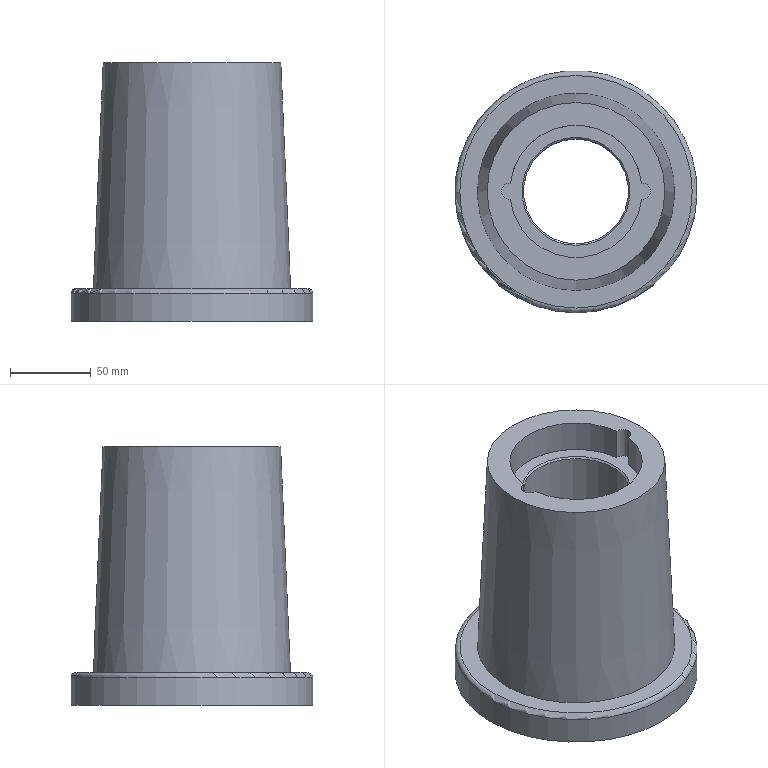Component | NX | BASE | 1 solid | 15 faces | box 150 x 150 x 160 mm | volume 816853 mm3 | cylinder 6 | plane 5 | cone 3 | torus 1 | commonest cylinder face diameters 82 x2 10 x2 150 x1 65 x1
STEP:
#1=CARTESIAN_POINT('',(0.,0.,0.));
#2=DIRECTION('',(0.,0.,1.));
#3=DIRECTION('',(1.,0.,0.));
#4=AXIS2_PLACEMENT_3D('',#1,#2,#3);
#5=CARTESIAN_POINT('',(-40.695,-4.991,140.));
#6=VERTEX_POINT('',#5);
#7=CARTESIAN_POINT('',(-40.695,-4.991,160.));
#8=VERTEX_POINT('',#7);
#9=CARTESIAN_POINT('',(-40.695,-4.991,150.));
#10=DIRECTION('',(0.,0.,1.));
#11=VECTOR('',#10,1.);
#12=LINE('',#9,#11);
#13=CARTESIAN_POINT('',(0.,0.,160.));
#14=DIRECTION('',(0.,0.,-1.));
#15=DIRECTION('',(0.,-1.,0.));
#16=AXIS2_PLACEMENT_3D('',#13,#14,#15);
#17=CYLINDRICAL_SURFACE('',#16,41.);
#18=CARTESIAN_POINT('',(1.449,10.));
#19=DIRECTION('',(0.,-1.));
#20=VECTOR('',#19,1.);
#21=LINE('',#18,#20);
#22=(GEOMETRIC_REPRESENTATION_CONTEXT(2)PARAMETRIC_REPRESENTATION_CONTEXT()REPRESENTATION_CONTEXT('',''));
#23=DEFINITIONAL_REPRESENTATION('',(#21),#22);
#24=PCURVE('',#17,#23);
#25=CARTESIAN_POINT('',(-41.,-0.,160.));
#26=DIRECTION('',(0.,0.,-1.));
#27=DIRECTION('',(0.,-1.,0.));
#28=AXIS2_PLACEMENT_3D('',#25,#26,#27);
#29=CYLINDRICAL_SURFACE('',#28,5.);
#30=CARTESIAN_POINT('',(-0.06101,10.));
#31=DIRECTION('',(0.,-1.));
#32=VECTOR('',#31,1.);
#33=LINE('',#30,#32);
#34=(GEOMETRIC_REPRESENTATION_CONTEXT(2)PARAMETRIC_REPRESENTATION_CONTEXT()REPRESENTATION_CONTEXT('',''));
#35=DEFINITIONAL_REPRESENTATION('',(#33),#34);
#36=PCURVE('',#29,#35);
#37=SURFACE_CURVE('',#12,(#24,#36),.PCURVE_S1.);
#38=EDGE_CURVE('',#6,#8,#37,.T.);
#39=ORIENTED_EDGE('',*,*,#38,.F.);
#40=CARTESIAN_POINT('',(40.695,-4.991,140.));
#41=VERTEX_POINT('',#40);
#42=CARTESIAN_POINT('',(0.,0.,140.));
#43=DIRECTION('',(0.,0.,-1.));
#44=DIRECTION('',(0.,-1.,0.));
#45=AXIS2_PLACEMENT_3D('',#42,#43,#44);
#46=CIRCLE('',#45,41.);
#47=CARTESIAN_POINT('',(-6.283,20.));
#48=DIRECTION('',(1.,0.));
#49=VECTOR('',#48,1.);
#50=LINE('',#47,#49);
#51=(GEOMETRIC_REPRESENTATION_CONTEXT(2)PARAMETRIC_REPRESENTATION_CONTEXT()REPRESENTATION_CONTEXT('',''));
#52=DEFINITIONAL_REPRESENTATION('',(#50),#51);
#53=PCURVE('',#17,#52);
#54=CARTESIAN_POINT('',(0.,0.,140.));
#55=DIRECTION('',(0.,0.,-1.));
#56=DIRECTION('',(0.,1.,0.));
#57=AXIS2_PLACEMENT_3D('',#54,#55,#56);
#58=PLANE('',#57);
#59=CARTESIAN_POINT('',(0.,0.));
#60=DIRECTION('',(-1.,0.));
#61=AXIS2_PLACEMENT_2D('',#59,#60);
#62=CIRCLE('',#61,41.);
#63=(GEOMETRIC_REPRESENTATION_CONTEXT(2)PARAMETRIC_REPRESENTATION_CONTEXT()REPRESENTATION_CONTEXT('',''));
#64=DEFINITIONAL_REPRESENTATION('',(#62),#63);
#65=PCURVE('',#58,#64);
#66=SURFACE_CURVE('',#46,(#53,#65),.PCURVE_S1.);
#67=EDGE_CURVE('',#41,#6,#66,.T.);
#68=ORIENTED_EDGE('',*,*,#67,.F.);
#69=CARTESIAN_POINT('',(40.695,-4.991,160.));
#70=VERTEX_POINT('',#69);
#71=CARTESIAN_POINT('',(40.695,-4.991,150.));
#72=DIRECTION('',(0.,0.,-1.));
#73=VECTOR('',#72,1.);
#74=LINE('',#71,#73);
#75=CARTESIAN_POINT('',(-1.449,10.));
#76=DIRECTION('',(0.,1.));
#77=VECTOR('',#76,1.);
#78=LINE('',#75,#77);
#79=(GEOMETRIC_REPRESENTATION_CONTEXT(2)PARAMETRIC_REPRESENTATION_CONTEXT()REPRESENTATION_CONTEXT('',''));
#80=DEFINITIONAL_REPRESENTATION('',(#78),#79);
#81=PCURVE('',#17,#80);
#82=CARTESIAN_POINT('',(41.,0.,160.));
#83=DIRECTION('',(0.,0.,-1.));
#84=DIRECTION('',(0.,-1.,0.));
#85=AXIS2_PLACEMENT_3D('',#82,#83,#84);
#86=CYLINDRICAL_SURFACE('',#85,5.);
#87=CARTESIAN_POINT('',(6.344,10.));
#88=DIRECTION('',(0.,1.));
#89=VECTOR('',#88,1.);
#90=LINE('',#87,#89);
#91=(GEOMETRIC_REPRESENTATION_CONTEXT(2)PARAMETRIC_REPRESENTATION_CONTEXT()REPRESENTATION_CONTEXT('',''));
#92=DEFINITIONAL_REPRESENTATION('',(#90),#91);
#93=PCURVE('',#86,#92);
#94=SURFACE_CURVE('',#74,(#81,#93),.PCURVE_S1.);
#95=EDGE_CURVE('',#70,#41,#94,.T.);
#96=ORIENTED_EDGE('',*,*,#95,.F.);
#97=CARTESIAN_POINT('',(0.,0.,160.));
#98=DIRECTION('',(0.,0.,-1.));
#99=DIRECTION('',(0.,-1.,0.));
#100=AXIS2_PLACEMENT_3D('',#97,#98,#99);
#101=CIRCLE('',#100,41.);
#102=CARTESIAN_POINT('',(-6.283,0.));
#103=DIRECTION('',(1.,0.));
#104=VECTOR('',#103,1.);
#105=LINE('',#102,#104);
#106=(GEOMETRIC_REPRESENTATION_CONTEXT(2)PARAMETRIC_REPRESENTATION_CONTEXT()REPRESENTATION_CONTEXT('',''));
#107=DEFINITIONAL_REPRESENTATION('',(#105),#106);
#108=PCURVE('',#17,#107);
#109=CARTESIAN_POINT('',(0.,0.,160.));
#110=DIRECTION('',(0.,0.,1.));
#111=DIRECTION('',(0.,-1.,0.));
#112=AXIS2_PLACEMENT_3D('',#109,#110,#111);
#113=PLANE('',#112);
#114=CARTESIAN_POINT('',(41.,0.));
#115=CARTESIAN_POINT('',(41.,-71.014));
#116=CARTESIAN_POINT('',(-20.5,-35.507));
#117=CARTESIAN_POINT('',(-82.,-0.));
#118=CARTESIAN_POINT('',(-20.5,35.507));
#119=CARTESIAN_POINT('',(41.,71.014));
#120=CARTESIAN_POINT('',(41.,0.));
#121=(BOUNDED_CURVE()B_SPLINE_CURVE(2,(#114,#115,#116,#117,#118,#119,#120),.UNSPECIFIED.,.T.,.F.)B_SPLINE_CURVE_WITH_KNOTS((1,2,2,2,2,1),(-2.094,0.,2.094,4.189,6.283,8.378),.UNSPECIFIED.)CURVE()GEOMETRIC_REPRESENTATION_ITEM()RATIONAL_B_SPLINE_CURVE((1.,0.5,1.,0.5,1.,0.5,1.))REPRESENTATION_ITEM(''));
#122=(GEOMETRIC_REPRESENTATION_CONTEXT(2)PARAMETRIC_REPRESENTATION_CONTEXT()REPRESENTATION_CONTEXT('',''));
#123=DEFINITIONAL_REPRESENTATION('',(#121),#122);
#124=PCURVE('',#113,#123);
#125=SURFACE_CURVE('',#101,(#108,#124),.PCURVE_S1.);
#126=EDGE_CURVE('',#70,#8,#125,.T.);
#127=ORIENTED_EDGE('',*,*,#126,.T.);
#128=EDGE_LOOP('',(#39,#68,#96,#127));
#129=FACE_BOUND('',#128,.F.);
#130=ADVANCED_FACE('',(#129),#17,.F.);
#131=CARTESIAN_POINT('',(0.,-61.113,20.));
#132=VERTEX_POINT('',#131);
#133=CARTESIAN_POINT('',(0.,0.,20.));
#134=DIRECTION('',(0.,0.,-1.));
#135=DIRECTION('',(0.,-1.,0.));
#136=AXIS2_PLACEMENT_3D('',#133,#134,#135);
#137=CIRCLE('',#136,61.113);
#138=CARTESIAN_POINT('',(0.,0.,160.));
#139=DIRECTION('',(0.,0.,-1.));
#140=DIRECTION('',(0.,-1.,0.));
#141=AXIS2_PLACEMENT_3D('',#138,#139,#140);
#142=CONICAL_SURFACE('',#141,55.,0.04363);
#143=CARTESIAN_POINT('',(0.,140.));
#144=DIRECTION('',(1.,0.));
#145=VECTOR('',#144,1.);
#146=LINE('',#143,#145);
#147=(GEOMETRIC_REPRESENTATION_CONTEXT(2)PARAMETRIC_REPRESENTATION_CONTEXT()REPRESENTATION_CONTEXT('',''));
#148=DEFINITIONAL_REPRESENTATION('',(#146),#147);
#149=PCURVE('',#142,#148);
#150=CARTESIAN_POINT('',(0.,0.,20.));
#151=DIRECTION('',(0.,0.,1.));
#152=DIRECTION('',(0.,-1.,0.));
#153=AXIS2_PLACEMENT_3D('',#150,#151,#152);
#154=PLANE('',#153);
#155=CARTESIAN_POINT('',(61.113,0.));
#156=CARTESIAN_POINT('',(61.113,-105.85));
#157=CARTESIAN_POINT('',(-30.556,-52.925));
#158=CARTESIAN_POINT('',(-122.225,-0.));
#159=CARTESIAN_POINT('',(-30.556,52.925));
#160=CARTESIAN_POINT('',(61.113,105.85));
#161=CARTESIAN_POINT('',(61.113,0.));
#162=(BOUNDED_CURVE()B_SPLINE_CURVE(2,(#155,#156,#157,#158,#159,#160,#161),.UNSPECIFIED.,.T.,.F.)B_SPLINE_CURVE_WITH_KNOTS((1,2,2,2,2,1),(-2.094,0.,2.094,4.189,6.283,8.378),.UNSPECIFIED.)CURVE()GEOMETRIC_REPRESENTATION_ITEM()RATIONAL_B_SPLINE_CURVE((1.,0.5,1.,0.5,1.,0.5,1.))REPRESENTATION_ITEM(''));
#163=(GEOMETRIC_REPRESENTATION_CONTEXT(2)PARAMETRIC_REPRESENTATION_CONTEXT()REPRESENTATION_CONTEXT('',''));
#164=DEFINITIONAL_REPRESENTATION('',(#162),#163);
#165=PCURVE('',#154,#164);
#166=SURFACE_CURVE('',#137,(#149,#165),.PCURVE_S1.);
#167=EDGE_CURVE('',#132,#132,#166,.T.);
#168=ORIENTED_EDGE('',*,*,#167,.F.);
#169=CARTESIAN_POINT('',(0.,-55.,160.));
#170=VERTEX_POINT('',#169);
#171=CARTESIAN_POINT('',(0.,-55.,160.));
#172=CARTESIAN_POINT('',(0.,-61.113,20.));
#173=B_SPLINE_CURVE_WITH_KNOTS('',1,(#171,#172),.UNSPECIFIED.,.F.,.F.,(2,2),(0.,140.133),.PIECEWISE_BEZIER_KNOTS.);
#174=CARTESIAN_POINT('',(0.,0.));
#175=DIRECTION('',(0.,1.));
#176=VECTOR('',#175,1.);
#177=LINE('',#174,#176);
#178=(GEOMETRIC_REPRESENTATION_CONTEXT(2)PARAMETRIC_REPRESENTATION_CONTEXT()REPRESENTATION_CONTEXT('',''));
#179=DEFINITIONAL_REPRESENTATION('',(#177),#178);
#180=PCURVE('',#142,#179);
#181=CARTESIAN_POINT('',(6.283,0.));
#182=DIRECTION('',(0.,1.));
#183=VECTOR('',#182,1.);
#184=LINE('',#181,#183);
#185=(GEOMETRIC_REPRESENTATION_CONTEXT(2)PARAMETRIC_REPRESENTATION_CONTEXT()REPRESENTATION_CONTEXT('',''));
#186=DEFINITIONAL_REPRESENTATION('',(#184),#185);
#187=PCURVE('',#142,#186);
#188=SEAM_CURVE('',#173,(#180,#187),.PCURVE_S1.);
#189=EDGE_CURVE('',#170,#132,#188,.T.);
#190=ORIENTED_EDGE('',*,*,#189,.F.);
#191=CARTESIAN_POINT('',(0.,0.,160.));
#192=DIRECTION('',(0.,0.,-1.));
#193=DIRECTION('',(0.,-1.,0.));
#194=AXIS2_PLACEMENT_3D('',#191,#192,#193);
#195=CIRCLE('',#194,55.);
#196=CARTESIAN_POINT('',(0.,0.));
#197=DIRECTION('',(1.,0.));
#198=VECTOR('',#197,1.);
#199=LINE('',#196,#198);
#200=(GEOMETRIC_REPRESENTATION_CONTEXT(2)PARAMETRIC_REPRESENTATION_CONTEXT()REPRESENTATION_CONTEXT('',''));
#201=DEFINITIONAL_REPRESENTATION('',(#199),#200);
#202=PCURVE('',#142,#201);
#203=CARTESIAN_POINT('',(55.,0.));
#204=CARTESIAN_POINT('',(55.,-95.263));
#205=CARTESIAN_POINT('',(-27.5,-47.631));
#206=CARTESIAN_POINT('',(-110.,-0.));
#207=CARTESIAN_POINT('',(-27.5,47.631));
#208=CARTESIAN_POINT('',(55.,95.263));
#209=CARTESIAN_POINT('',(55.,0.));
#210=(BOUNDED_CURVE()B_SPLINE_CURVE(2,(#203,#204,#205,#206,#207,#208,#209),.UNSPECIFIED.,.T.,.F.)B_SPLINE_CURVE_WITH_KNOTS((1,2,2,2,2,1),(-2.094,0.,2.094,4.189,6.283,8.378),.UNSPECIFIED.)CURVE()GEOMETRIC_REPRESENTATION_ITEM()RATIONAL_B_SPLINE_CURVE((1.,0.5,1.,0.5,1.,0.5,1.))REPRESENTATION_ITEM(''));
#211=(GEOMETRIC_REPRESENTATION_CONTEXT(2)PARAMETRIC_REPRESENTATION_CONTEXT()REPRESENTATION_CONTEXT('',''));
#212=DEFINITIONAL_REPRESENTATION('',(#210),#211);
#213=PCURVE('',#113,#212);
#214=SURFACE_CURVE('',#195,(#202,#213),.PCURVE_S1.);
#215=EDGE_CURVE('',#170,#170,#214,.T.);
#216=ORIENTED_EDGE('',*,*,#215,.T.);
#217=ORIENTED_EDGE('',*,*,#189,.T.);
#218=EDGE_LOOP('',(#168,#190,#216,#217));
#219=FACE_BOUND('',#218,.T.);
#220=ADVANCED_FACE('',(#219),#142,.T.);
#221=CARTESIAN_POINT('',(0.,-51.976,-0.));
#222=VERTEX_POINT('',#221);
#223=CARTESIAN_POINT('',(0.,51.976,0.));
#224=VERTEX_POINT('',#223);
#225=CARTESIAN_POINT('',(0.,0.,0.));
#226=DIRECTION('',(0.,0.,-1.));
#227=DIRECTION('',(0.,1.,0.));
#228=AXIS2_PLACEMENT_3D('',#225,#226,#227);
#229=CIRCLE('',#228,51.976);
#230=CARTESIAN_POINT('',(0.,0.,159.564));
#231=DIRECTION('',(0.,0.,-1.));
#232=DIRECTION('',(0.,-1.,0.));
#233=AXIS2_PLACEMENT_3D('',#230,#231,#232);
#234=CONICAL_SURFACE('',#233,45.01,0.04363);
#235=CARTESIAN_POINT('',(-3.142,159.564));
#236=DIRECTION('',(1.,0.));
#237=VECTOR('',#236,1.);
#238=LINE('',#235,#237);
#239=(GEOMETRIC_REPRESENTATION_CONTEXT(2)PARAMETRIC_REPRESENTATION_CONTEXT()REPRESENTATION_CONTEXT('',''));
#240=DEFINITIONAL_REPRESENTATION('',(#238),#239);
#241=PCURVE('',#234,#240);
#242=CARTESIAN_POINT('',(0.,0.,0.));
#243=DIRECTION('',(0.,0.,-1.));
#244=DIRECTION('',(0.,1.,0.));
#245=AXIS2_PLACEMENT_3D('',#242,#243,#244);
#246=PLANE('',#245);
#247=CARTESIAN_POINT('',(0.,0.));
#248=DIRECTION('',(1.,0.));
#249=AXIS2_PLACEMENT_2D('',#247,#248);
#250=CIRCLE('',#249,51.976);
#251=(GEOMETRIC_REPRESENTATION_CONTEXT(2)PARAMETRIC_REPRESENTATION_CONTEXT()REPRESENTATION_CONTEXT('',''));
#252=DEFINITIONAL_REPRESENTATION('',(#250),#251);
#253=PCURVE('',#246,#252);
#254=SURFACE_CURVE('',#229,(#241,#253),.PCURVE_S1.);
#255=EDGE_CURVE('',#222,#224,#254,.T.);
#256=ORIENTED_EDGE('',*,*,#255,.F.);
#257=CARTESIAN_POINT('',(0.,-47.61,100.));
#258=VERTEX_POINT('',#257);
#259=CARTESIAN_POINT('',(0.,-47.61,100.));
#260=CARTESIAN_POINT('',(0.,-51.976,-0.));
#261=B_SPLINE_CURVE_WITH_KNOTS('',1,(#259,#260),.UNSPECIFIED.,.F.,.F.,(2,2),(59.621,159.716),.PIECEWISE_BEZIER_KNOTS.);
#262=CARTESIAN_POINT('',(0.,0.));
#263=DIRECTION('',(0.,1.));
#264=VECTOR('',#263,1.);
#265=LINE('',#262,#264);
#266=(GEOMETRIC_REPRESENTATION_CONTEXT(2)PARAMETRIC_REPRESENTATION_CONTEXT()REPRESENTATION_CONTEXT('',''));
#267=DEFINITIONAL_REPRESENTATION('',(#265),#266);
#268=PCURVE('',#234,#267);
#269=CARTESIAN_POINT('',(6.283,0.));
#270=DIRECTION('',(0.,1.));
#271=VECTOR('',#270,1.);
#272=LINE('',#269,#271);
#273=(GEOMETRIC_REPRESENTATION_CONTEXT(2)PARAMETRIC_REPRESENTATION_CONTEXT()REPRESENTATION_CONTEXT('',''));
#274=DEFINITIONAL_REPRESENTATION('',(#272),#273);
#275=PCURVE('',#234,#274);
#276=SEAM_CURVE('',#261,(#268,#275),.PCURVE_S1.);
#277=EDGE_CURVE('',#258,#222,#276,.T.);
#278=ORIENTED_EDGE('',*,*,#277,.F.);
#279=CARTESIAN_POINT('',(0.,0.,100.));
#280=DIRECTION('',(0.,0.,-1.));
#281=DIRECTION('',(0.,-1.,0.));
#282=AXIS2_PLACEMENT_3D('',#279,#280,#281);
#283=CIRCLE('',#282,47.61);
#284=CARTESIAN_POINT('',(0.,59.564));
#285=DIRECTION('',(1.,0.));
#286=VECTOR('',#285,1.);
#287=LINE('',#284,#286);
#288=(GEOMETRIC_REPRESENTATION_CONTEXT(2)PARAMETRIC_REPRESENTATION_CONTEXT()REPRESENTATION_CONTEXT('',''));
#289=DEFINITIONAL_REPRESENTATION('',(#287),#288);
#290=PCURVE('',#234,#289);
#291=CARTESIAN_POINT('',(0.,0.,100.));
#292=DIRECTION('',(0.,0.,1.));
#293=DIRECTION('',(0.,-1.,0.));
#294=AXIS2_PLACEMENT_3D('',#291,#292,#293);
#295=PLANE('',#294);
#296=CARTESIAN_POINT('',(47.61,0.));
#297=CARTESIAN_POINT('',(47.61,-82.463));
#298=CARTESIAN_POINT('',(-23.805,-41.232));
#299=CARTESIAN_POINT('',(-95.22,-0.));
#300=CARTESIAN_POINT('',(-23.805,41.232));
#301=CARTESIAN_POINT('',(47.61,82.463));
#302=CARTESIAN_POINT('',(47.61,0.));
#303=(BOUNDED_CURVE()B_SPLINE_CURVE(2,(#296,#297,#298,#299,#300,#301,#302),.UNSPECIFIED.,.T.,.F.)B_SPLINE_CURVE_WITH_KNOTS((1,2,2,2,2,1),(-2.094,0.,2.094,4.189,6.283,8.378),.UNSPECIFIED.)CURVE()GEOMETRIC_REPRESENTATION_ITEM()RATIONAL_B_SPLINE_CURVE((1.,0.5,1.,0.5,1.,0.5,1.))REPRESENTATION_ITEM(''));
#304=(GEOMETRIC_REPRESENTATION_CONTEXT(2)PARAMETRIC_REPRESENTATION_CONTEXT()REPRESENTATION_CONTEXT('',''));
#305=DEFINITIONAL_REPRESENTATION('',(#303),#304);
#306=PCURVE('',#295,#305);
#307=SURFACE_CURVE('',#283,(#290,#306),.PCURVE_S1.);
#308=EDGE_CURVE('',#258,#258,#307,.T.);
#309=ORIENTED_EDGE('',*,*,#308,.T.);
#310=ORIENTED_EDGE('',*,*,#277,.T.);
#311=CARTESIAN_POINT('',(0.,0.,0.));
#312=DIRECTION('',(0.,0.,-1.));
#313=DIRECTION('',(0.,1.,0.));
#314=AXIS2_PLACEMENT_3D('',#311,#312,#313);
#315=CIRCLE('',#314,51.976);
#316=CARTESIAN_POINT('',(3.142,159.564));
#317=DIRECTION('',(1.,0.));
#318=VECTOR('',#317,1.);
#319=LINE('',#316,#318);
#320=(GEOMETRIC_REPRESENTATION_CONTEXT(2)PARAMETRIC_REPRESENTATION_CONTEXT()REPRESENTATION_CONTEXT('',''));
#321=DEFINITIONAL_REPRESENTATION('',(#319),#320);
#322=PCURVE('',#234,#321);
#323=CARTESIAN_POINT('',(0.,0.));
#324=DIRECTION('',(1.,0.));
#325=AXIS2_PLACEMENT_2D('',#323,#324);
#326=CIRCLE('',#325,51.976);
#327=(GEOMETRIC_REPRESENTATION_CONTEXT(2)PARAMETRIC_REPRESENTATION_CONTEXT()REPRESENTATION_CONTEXT('',''));
#328=DEFINITIONAL_REPRESENTATION('',(#326),#327);
#329=PCURVE('',#246,#328);
#330=SURFACE_CURVE('',#315,(#322,#329),.PCURVE_S1.);
#331=EDGE_CURVE('',#224,#222,#330,.T.);
#332=ORIENTED_EDGE('',*,*,#331,.F.);
#333=EDGE_LOOP('',(#256,#278,#309,#310,#332));
#334=FACE_BOUND('',#333,.F.);
#335=ADVANCED_FACE('',(#334),#234,.F.);
#336=CARTESIAN_POINT('',(0.,-72.,20.));
#337=VERTEX_POINT('',#336);
#338=CARTESIAN_POINT('',(0.,0.,20.));
#339=DIRECTION('',(0.,0.,1.));
#340=DIRECTION('',(0.,-1.,0.));
#341=AXIS2_PLACEMENT_3D('',#338,#339,#340);
#342=CIRCLE('',#341,72.);
#343=CARTESIAN_POINT('',(0.,0.));
#344=DIRECTION('',(1.,0.));
#345=AXIS2_PLACEMENT_2D('',#343,#344);
#346=CIRCLE('',#345,72.);
#347=(GEOMETRIC_REPRESENTATION_CONTEXT(2)PARAMETRIC_REPRESENTATION_CONTEXT()REPRESENTATION_CONTEXT('',''));
#348=DEFINITIONAL_REPRESENTATION('',(#346),#347);
#349=PCURVE('',#154,#348);
#350=CARTESIAN_POINT('',(0.,0.,17.));
#351=DIRECTION('',(0.,0.,1.));
#352=DIRECTION('',(0.,-1.,0.));
#353=AXIS2_PLACEMENT_3D('',#350,#351,#352);
#354=TOROIDAL_SURFACE('',#353,72.,3.);
#355=CARTESIAN_POINT('',(0.,7.854));
#356=DIRECTION('',(1.,0.));
#357=VECTOR('',#356,1.);
#358=LINE('',#355,#357);
#359=(GEOMETRIC_REPRESENTATION_CONTEXT(2)PARAMETRIC_REPRESENTATION_CONTEXT()REPRESENTATION_CONTEXT('',''));
#360=DEFINITIONAL_REPRESENTATION('',(#358),#359);
#361=PCURVE('',#354,#360);
#362=SURFACE_CURVE('',#342,(#349,#361),.PCURVE_S1.);
#363=EDGE_CURVE('',#337,#337,#362,.T.);
#364=ORIENTED_EDGE('',*,*,#363,.T.);
#365=EDGE_LOOP('',(#364));
#366=FACE_BOUND('',#365,.T.);
#367=ORIENTED_EDGE('',*,*,#167,.T.);
#368=EDGE_LOOP('',(#367));
#369=FACE_BOUND('',#368,.T.);
#370=ADVANCED_FACE('',(#366,#369),#154,.T.);
#371=CARTESIAN_POINT('',(0.,-75.,17.));
#372=VERTEX_POINT('',#371);
#373=CARTESIAN_POINT('',(0.,0.,17.));
#374=DIRECTION('',(0.,0.,-1.));
#375=DIRECTION('',(0.,-1.,0.));
#376=AXIS2_PLACEMENT_3D('',#373,#374,#375);
#377=CIRCLE('',#376,75.);
#378=CARTESIAN_POINT('',(0.,0.,0.));
#379=DIRECTION('',(0.,0.,1.));
#380=DIRECTION('',(0.,-1.,0.));
#381=AXIS2_PLACEMENT_3D('',#378,#379,#380);
#382=CYLINDRICAL_SURFACE('',#381,75.);
#383=CARTESIAN_POINT('',(6.283,17.));
#384=DIRECTION('',(-1.,0.));
#385=VECTOR('',#384,1.);
#386=LINE('',#383,#385);
#387=(GEOMETRIC_REPRESENTATION_CONTEXT(2)PARAMETRIC_REPRESENTATION_CONTEXT()REPRESENTATION_CONTEXT('',''));
#388=DEFINITIONAL_REPRESENTATION('',(#386),#387);
#389=PCURVE('',#382,#388);
#390=CARTESIAN_POINT('',(6.283,6.283));
#391=DIRECTION('',(-1.,0.));
#392=VECTOR('',#391,1.);
#393=LINE('',#390,#392);
#394=(GEOMETRIC_REPRESENTATION_CONTEXT(2)PARAMETRIC_REPRESENTATION_CONTEXT()REPRESENTATION_CONTEXT('',''));
#395=DEFINITIONAL_REPRESENTATION('',(#393),#394);
#396=PCURVE('',#354,#395);
#397=SURFACE_CURVE('',#377,(#389,#396),.PCURVE_S1.);
#398=EDGE_CURVE('',#372,#372,#397,.T.);
#399=ORIENTED_EDGE('',*,*,#398,.T.);
#400=CARTESIAN_POINT('',(0.,-75.,0.));
#401=VERTEX_POINT('',#400);
#402=CARTESIAN_POINT('',(-0.,-75.,0.));
#403=CARTESIAN_POINT('',(-0.,-75.,17.));
#404=B_SPLINE_CURVE_WITH_KNOTS('',1,(#402,#403),.UNSPECIFIED.,.F.,.F.,(2,2),(0.,17.),.PIECEWISE_BEZIER_KNOTS.);
#405=CARTESIAN_POINT('',(0.,0.));
#406=DIRECTION('',(0.,1.));
#407=VECTOR('',#406,1.);
#408=LINE('',#405,#407);
#409=(GEOMETRIC_REPRESENTATION_CONTEXT(2)PARAMETRIC_REPRESENTATION_CONTEXT()REPRESENTATION_CONTEXT('',''));
#410=DEFINITIONAL_REPRESENTATION('',(#408),#409);
#411=PCURVE('',#382,#410);
#412=CARTESIAN_POINT('',(6.283,0.));
#413=DIRECTION('',(0.,1.));
#414=VECTOR('',#413,1.);
#415=LINE('',#412,#414);
#416=(GEOMETRIC_REPRESENTATION_CONTEXT(2)PARAMETRIC_REPRESENTATION_CONTEXT()REPRESENTATION_CONTEXT('',''));
#417=DEFINITIONAL_REPRESENTATION('',(#415),#416);
#418=PCURVE('',#382,#417);
#419=SEAM_CURVE('',#404,(#411,#418),.PCURVE_S1.);
#420=EDGE_CURVE('',#401,#372,#419,.T.);
#421=ORIENTED_EDGE('',*,*,#420,.F.);
#422=CARTESIAN_POINT('',(0.,0.,0.));
#423=DIRECTION('',(0.,0.,1.));
#424=DIRECTION('',(0.,-1.,0.));
#425=AXIS2_PLACEMENT_3D('',#422,#423,#424);
#426=CIRCLE('',#425,75.);
#427=CARTESIAN_POINT('',(0.,0.));
#428=DIRECTION('',(1.,0.));
#429=VECTOR('',#428,1.);
#430=LINE('',#427,#429);
#431=(GEOMETRIC_REPRESENTATION_CONTEXT(2)PARAMETRIC_REPRESENTATION_CONTEXT()REPRESENTATION_CONTEXT('',''));
#432=DEFINITIONAL_REPRESENTATION('',(#430),#431);
#433=PCURVE('',#382,#432);
#434=CARTESIAN_POINT('',(-75.,0.));
#435=CARTESIAN_POINT('',(-75.,129.904));
#436=CARTESIAN_POINT('',(37.5,64.952));
#437=CARTESIAN_POINT('',(150.,0.));
#438=CARTESIAN_POINT('',(37.5,-64.952));
#439=CARTESIAN_POINT('',(-75.,-129.904));
#440=CARTESIAN_POINT('',(-75.,0.));
#441=(BOUNDED_CURVE()B_SPLINE_CURVE(2,(#434,#435,#436,#437,#438,#439,#440),.UNSPECIFIED.,.T.,.F.)B_SPLINE_CURVE_WITH_KNOTS((1,2,2,2,2,1),(-2.094,0.,2.094,4.189,6.283,8.378),.UNSPECIFIED.)CURVE()GEOMETRIC_REPRESENTATION_ITEM()RATIONAL_B_SPLINE_CURVE((1.,0.5,1.,0.5,1.,0.5,1.))REPRESENTATION_ITEM(''));
#442=(GEOMETRIC_REPRESENTATION_CONTEXT(2)PARAMETRIC_REPRESENTATION_CONTEXT()REPRESENTATION_CONTEXT('',''));
#443=DEFINITIONAL_REPRESENTATION('',(#441),#442);
#444=PCURVE('',#246,#443);
#445=SURFACE_CURVE('',#426,(#433,#444),.PCURVE_S1.);
#446=EDGE_CURVE('',#401,#401,#445,.T.);
#447=ORIENTED_EDGE('',*,*,#446,.T.);
#448=ORIENTED_EDGE('',*,*,#420,.T.);
#449=EDGE_LOOP('',(#399,#421,#447,#448));
#450=FACE_BOUND('',#449,.T.);
#451=ADVANCED_FACE('',(#450),#382,.T.);
#452=ORIENTED_EDGE('',*,*,#446,.F.);
#453=EDGE_LOOP('',(#452));
#454=FACE_BOUND('',#453,.T.);
#455=ORIENTED_EDGE('',*,*,#331,.F.);
#456=ORIENTED_EDGE('',*,*,#255,.F.);
#457=EDGE_LOOP('',(#455,#456));
#458=FACE_BOUND('',#457,.T.);
#459=ADVANCED_FACE('',(#454,#458),#246,.T.);
#460=ORIENTED_EDGE('',*,*,#363,.F.);
#461=CARTESIAN_POINT('',(-0.,-75.,17.));
#462=CARTESIAN_POINT('',(-0.,-75.,17.802));
#463=CARTESIAN_POINT('',(-0.,-74.745,18.583));
#464=CARTESIAN_POINT('',(-0.,-74.256,19.256));
#465=CARTESIAN_POINT('',(-0.,-73.583,19.745));
#466=CARTESIAN_POINT('',(-0.,-72.802,20.));
#467=CARTESIAN_POINT('',(-0.,-72.,20.));
#468=(BOUNDED_CURVE()B_SPLINE_CURVE(6,(#461,#462,#463,#464,#465,#466,#467),.UNSPECIFIED.,.F.,.F.)B_SPLINE_CURVE_WITH_KNOTS((7,7),(0.,1.571),.PIECEWISE_BEZIER_KNOTS.)CURVE()GEOMETRIC_REPRESENTATION_ITEM()RATIONAL_B_SPLINE_CURVE((1.031,1.01,0.9979,0.994,0.9979,1.01,1.031))REPRESENTATION_ITEM(''));
#469=CARTESIAN_POINT('',(0.,6.283));
#470=DIRECTION('',(0.,1.));
#471=VECTOR('',#470,1.);
#472=LINE('',#469,#471);
#473=(GEOMETRIC_REPRESENTATION_CONTEXT(2)PARAMETRIC_REPRESENTATION_CONTEXT()REPRESENTATION_CONTEXT('',''));
#474=DEFINITIONAL_REPRESENTATION('',(#472),#473);
#475=PCURVE('',#354,#474);
#476=CARTESIAN_POINT('',(6.283,6.283));
#477=DIRECTION('',(0.,1.));
#478=VECTOR('',#477,1.);
#479=LINE('',#476,#478);
#480=(GEOMETRIC_REPRESENTATION_CONTEXT(2)PARAMETRIC_REPRESENTATION_CONTEXT()REPRESENTATION_CONTEXT('',''));
#481=DEFINITIONAL_REPRESENTATION('',(#479),#480);
#482=PCURVE('',#354,#481);
#483=SEAM_CURVE('',#468,(#475,#482),.PCURVE_S1.);
#484=EDGE_CURVE('',#372,#337,#483,.T.);
#485=ORIENTED_EDGE('',*,*,#484,.F.);
#486=ORIENTED_EDGE('',*,*,#398,.F.);
#487=ORIENTED_EDGE('',*,*,#484,.T.);
#488=EDGE_LOOP('',(#460,#485,#486,#487));
#489=FACE_BOUND('',#488,.T.);
#490=ADVANCED_FACE('',(#489),#354,.T.);
#491=CARTESIAN_POINT('',(0.,-32.5,100.));
#492=VERTEX_POINT('',#491);
#493=CARTESIAN_POINT('',(0.,0.,100.));
#494=DIRECTION('',(0.,0.,1.));
#495=DIRECTION('',(0.,-1.,0.));
#496=AXIS2_PLACEMENT_3D('',#493,#494,#495);
#497=CIRCLE('',#496,32.5);
#498=CARTESIAN_POINT('',(0.,0.));
#499=DIRECTION('',(1.,0.));
#500=AXIS2_PLACEMENT_2D('',#498,#499);
#501=CIRCLE('',#500,32.5);
#502=(GEOMETRIC_REPRESENTATION_CONTEXT(2)PARAMETRIC_REPRESENTATION_CONTEXT()REPRESENTATION_CONTEXT('',''));
#503=DEFINITIONAL_REPRESENTATION('',(#501),#502);
#504=PCURVE('',#295,#503);
#505=CARTESIAN_POINT('',(0.,0.,160.));
#506=DIRECTION('',(0.,0.,-1.));
#507=DIRECTION('',(0.,-1.,0.));
#508=AXIS2_PLACEMENT_3D('',#505,#506,#507);
#509=CYLINDRICAL_SURFACE('',#508,32.5);
#510=CARTESIAN_POINT('',(6.283,60.));
#511=DIRECTION('',(-1.,0.));
#512=VECTOR('',#511,1.);
#513=LINE('',#510,#512);
#514=(GEOMETRIC_REPRESENTATION_CONTEXT(2)PARAMETRIC_REPRESENTATION_CONTEXT()REPRESENTATION_CONTEXT('',''));
#515=DEFINITIONAL_REPRESENTATION('',(#513),#514);
#516=PCURVE('',#509,#515);
#517=SURFACE_CURVE('',#497,(#504,#516),.PCURVE_S1.);
#518=EDGE_CURVE('',#492,#492,#517,.T.);
#519=ORIENTED_EDGE('',*,*,#518,.T.);
#520=EDGE_LOOP('',(#519));
#521=FACE_BOUND('',#520,.T.);
#522=ORIENTED_EDGE('',*,*,#308,.T.);
#523=EDGE_LOOP('',(#522));
#524=FACE_BOUND('',#523,.T.);
#525=ADVANCED_FACE('',(#521,#524),#295,.F.);
#526=CARTESIAN_POINT('',(40.695,4.991,160.));
#527=VERTEX_POINT('',#526);
#528=CARTESIAN_POINT('',(41.,0.,160.));
#529=DIRECTION('',(0.,0.,-1.));
#530=DIRECTION('',(0.,-1.,0.));
#531=AXIS2_PLACEMENT_3D('',#528,#529,#530);
#532=CIRCLE('',#531,5.);
#533=CARTESIAN_POINT('',(5.,41.));
#534=CARTESIAN_POINT('',(5.,32.34));
#535=CARTESIAN_POINT('',(-2.5,36.67));
#536=CARTESIAN_POINT('',(-10.,41.));
#537=CARTESIAN_POINT('',(-2.5,45.33));
#538=CARTESIAN_POINT('',(5.,49.66));
#539=CARTESIAN_POINT('',(5.,41.));
#540=(BOUNDED_CURVE()B_SPLINE_CURVE(2,(#533,#534,#535,#536,#537,#538,#539),.UNSPECIFIED.,.T.,.F.)B_SPLINE_CURVE_WITH_KNOTS((1,2,2,2,2,1),(-2.094,0.,2.094,4.189,6.283,8.378),.UNSPECIFIED.)CURVE()GEOMETRIC_REPRESENTATION_ITEM()RATIONAL_B_SPLINE_CURVE((1.,0.5,1.,0.5,1.,0.5,1.))REPRESENTATION_ITEM(''));
#541=(GEOMETRIC_REPRESENTATION_CONTEXT(2)PARAMETRIC_REPRESENTATION_CONTEXT()REPRESENTATION_CONTEXT('',''));
#542=DEFINITIONAL_REPRESENTATION('',(#540),#541);
#543=PCURVE('',#113,#542);
#544=CARTESIAN_POINT('',(0.,0.));
#545=DIRECTION('',(1.,0.));
#546=VECTOR('',#545,1.);
#547=LINE('',#544,#546);
#548=(GEOMETRIC_REPRESENTATION_CONTEXT(2)PARAMETRIC_REPRESENTATION_CONTEXT()REPRESENTATION_CONTEXT('',''));
#549=DEFINITIONAL_REPRESENTATION('',(#547),#548);
#550=PCURVE('',#86,#549);
#551=SURFACE_CURVE('',#532,(#543,#550),.PCURVE_S1.);
#552=EDGE_CURVE('',#527,#70,#551,.T.);
#553=ORIENTED_EDGE('',*,*,#552,.T.);
#554=ORIENTED_EDGE('',*,*,#126,.T.);
#555=CARTESIAN_POINT('',(-40.695,4.991,160.));
#556=VERTEX_POINT('',#555);
#557=CARTESIAN_POINT('',(-41.,-0.,160.));
#558=DIRECTION('',(0.,0.,-1.));
#559=DIRECTION('',(0.,-1.,0.));
#560=AXIS2_PLACEMENT_3D('',#557,#558,#559);
#561=CIRCLE('',#560,5.);
#562=CARTESIAN_POINT('',(5.,-41.));
#563=CARTESIAN_POINT('',(5.,-49.66));
#564=CARTESIAN_POINT('',(-2.5,-45.33));
#565=CARTESIAN_POINT('',(-10.,-41.));
#566=CARTESIAN_POINT('',(-2.5,-36.67));
#567=CARTESIAN_POINT('',(5.,-32.34));
#568=CARTESIAN_POINT('',(5.,-41.));
#569=(BOUNDED_CURVE()B_SPLINE_CURVE(2,(#562,#563,#564,#565,#566,#567,#568),.UNSPECIFIED.,.T.,.F.)B_SPLINE_CURVE_WITH_KNOTS((1,2,2,2,2,1),(-2.094,0.,2.094,4.189,6.283,8.378),.UNSPECIFIED.)CURVE()GEOMETRIC_REPRESENTATION_ITEM()RATIONAL_B_SPLINE_CURVE((1.,0.5,1.,0.5,1.,0.5,1.))REPRESENTATION_ITEM(''));
#570=(GEOMETRIC_REPRESENTATION_CONTEXT(2)PARAMETRIC_REPRESENTATION_CONTEXT()REPRESENTATION_CONTEXT('',''));
#571=DEFINITIONAL_REPRESENTATION('',(#569),#570);
#572=PCURVE('',#113,#571);
#573=CARTESIAN_POINT('',(-6.283,0.));
#574=DIRECTION('',(1.,0.));
#575=VECTOR('',#574,1.);
#576=LINE('',#573,#575);
#577=(GEOMETRIC_REPRESENTATION_CONTEXT(2)PARAMETRIC_REPRESENTATION_CONTEXT()REPRESENTATION_CONTEXT('',''));
#578=DEFINITIONAL_REPRESENTATION('',(#576),#577);
#579=PCURVE('',#29,#578);
#580=SURFACE_CURVE('',#561,(#572,#579),.PCURVE_S1.);
#581=EDGE_CURVE('',#8,#556,#580,.T.);
#582=ORIENTED_EDGE('',*,*,#581,.T.);
#583=CARTESIAN_POINT('',(0.,0.,160.));
#584=DIRECTION('',(0.,0.,-1.));
#585=DIRECTION('',(0.,-1.,0.));
#586=AXIS2_PLACEMENT_3D('',#583,#584,#585);
#587=CIRCLE('',#586,41.);
#588=CARTESIAN_POINT('',(41.,0.));
#589=CARTESIAN_POINT('',(41.,-71.014));
#590=CARTESIAN_POINT('',(-20.5,-35.507));
#591=CARTESIAN_POINT('',(-82.,-0.));
#592=CARTESIAN_POINT('',(-20.5,35.507));
#593=CARTESIAN_POINT('',(41.,71.014));
#594=CARTESIAN_POINT('',(41.,0.));
#595=(BOUNDED_CURVE()B_SPLINE_CURVE(2,(#588,#589,#590,#591,#592,#593,#594),.UNSPECIFIED.,.T.,.F.)B_SPLINE_CURVE_WITH_KNOTS((1,2,2,2,2,1),(-2.094,0.,2.094,4.189,6.283,8.378),.UNSPECIFIED.)CURVE()GEOMETRIC_REPRESENTATION_ITEM()RATIONAL_B_SPLINE_CURVE((1.,0.5,1.,0.5,1.,0.5,1.))REPRESENTATION_ITEM(''));
#596=(GEOMETRIC_REPRESENTATION_CONTEXT(2)PARAMETRIC_REPRESENTATION_CONTEXT()REPRESENTATION_CONTEXT('',''));
#597=DEFINITIONAL_REPRESENTATION('',(#595),#596);
#598=PCURVE('',#113,#597);
#599=CARTESIAN_POINT('',(0.,0.,160.));
#600=DIRECTION('',(0.,0.,-1.));
#601=DIRECTION('',(0.,-1.,0.));
#602=AXIS2_PLACEMENT_3D('',#599,#600,#601);
#603=CYLINDRICAL_SURFACE('',#602,41.);
#604=CARTESIAN_POINT('',(0.,0.));
#605=DIRECTION('',(1.,0.));
#606=VECTOR('',#605,1.);
#607=LINE('',#604,#606);
#608=(GEOMETRIC_REPRESENTATION_CONTEXT(2)PARAMETRIC_REPRESENTATION_CONTEXT()REPRESENTATION_CONTEXT('',''));
#609=DEFINITIONAL_REPRESENTATION('',(#607),#608);
#610=PCURVE('',#603,#609);
#611=SURFACE_CURVE('',#587,(#598,#610),.PCURVE_S1.);
#612=EDGE_CURVE('',#556,#527,#611,.T.);
#613=ORIENTED_EDGE('',*,*,#612,.T.);
#614=EDGE_LOOP('',(#553,#554,#582,#613));
#615=FACE_BOUND('',#614,.T.);
#616=ORIENTED_EDGE('',*,*,#215,.F.);
#617=EDGE_LOOP('',(#616));
#618=FACE_BOUND('',#617,.T.);
#619=ADVANCED_FACE('',(#615,#618),#113,.T.);
#620=CARTESIAN_POINT('',(0.,-32.5,139.));
#621=VERTEX_POINT('',#620);
#622=CARTESIAN_POINT('',(0.,32.5,139.));
#623=VERTEX_POINT('',#622);
#624=CARTESIAN_POINT('',(0.,0.,139.));
#625=DIRECTION('',(0.,0.,1.));
#626=DIRECTION('',(0.,1.,0.));
#627=AXIS2_PLACEMENT_3D('',#624,#625,#626);
#628=CIRCLE('',#627,32.5);
#629=CARTESIAN_POINT('',(9.425,21.));
#630=DIRECTION('',(-1.,0.));
#631=VECTOR('',#630,1.);
#632=LINE('',#629,#631);
#633=(GEOMETRIC_REPRESENTATION_CONTEXT(2)PARAMETRIC_REPRESENTATION_CONTEXT()REPRESENTATION_CONTEXT('',''));
#634=DEFINITIONAL_REPRESENTATION('',(#632),#633);
#635=PCURVE('',#509,#634);
#636=CARTESIAN_POINT('',(0.,0.,139.));
#637=DIRECTION('',(0.,0.,1.));
#638=DIRECTION('',(0.,-1.,0.));
#639=AXIS2_PLACEMENT_3D('',#636,#637,#638);
#640=CONICAL_SURFACE('',#639,32.5,0.7854);
#641=CARTESIAN_POINT('',(3.142,0.));
#642=DIRECTION('',(1.,0.));
#643=VECTOR('',#642,1.);
#644=LINE('',#641,#643);
#645=(GEOMETRIC_REPRESENTATION_CONTEXT(2)PARAMETRIC_REPRESENTATION_CONTEXT()REPRESENTATION_CONTEXT('',''));
#646=DEFINITIONAL_REPRESENTATION('',(#644),#645);
#647=PCURVE('',#640,#646);
#648=SURFACE_CURVE('',#628,(#635,#647),.PCURVE_S1.);
#649=EDGE_CURVE('',#621,#623,#648,.T.);
#650=ORIENTED_EDGE('',*,*,#649,.F.);
#651=CARTESIAN_POINT('',(0.,-32.5,139.));
#652=CARTESIAN_POINT('',(0.,-32.5,100.));
#653=B_SPLINE_CURVE_WITH_KNOTS('',1,(#651,#652),.UNSPECIFIED.,.F.,.F.,(2,2),(21.,60.),.PIECEWISE_BEZIER_KNOTS.);
#654=CARTESIAN_POINT('',(6.283,0.));
#655=DIRECTION('',(0.,1.));
#656=VECTOR('',#655,1.);
#657=LINE('',#654,#656);
#658=(GEOMETRIC_REPRESENTATION_CONTEXT(2)PARAMETRIC_REPRESENTATION_CONTEXT()REPRESENTATION_CONTEXT('',''));
#659=DEFINITIONAL_REPRESENTATION('',(#657),#658);
#660=PCURVE('',#509,#659);
#661=CARTESIAN_POINT('',(0.,0.));
#662=DIRECTION('',(0.,1.));
#663=VECTOR('',#662,1.);
#664=LINE('',#661,#663);
#665=(GEOMETRIC_REPRESENTATION_CONTEXT(2)PARAMETRIC_REPRESENTATION_CONTEXT()REPRESENTATION_CONTEXT('',''));
#666=DEFINITIONAL_REPRESENTATION('',(#664),#665);
#667=PCURVE('',#509,#666);
#668=SEAM_CURVE('',#653,(#660,#667),.PCURVE_S1.);
#669=EDGE_CURVE('',#621,#492,#668,.T.);
#670=ORIENTED_EDGE('',*,*,#669,.T.);
#671=ORIENTED_EDGE('',*,*,#518,.T.);
#672=ORIENTED_EDGE('',*,*,#669,.F.);
#673=CARTESIAN_POINT('',(0.,0.,139.));
#674=DIRECTION('',(0.,0.,1.));
#675=DIRECTION('',(0.,1.,0.));
#676=AXIS2_PLACEMENT_3D('',#673,#674,#675);
#677=CIRCLE('',#676,32.5);
#678=CARTESIAN_POINT('',(3.142,21.));
#679=DIRECTION('',(-1.,0.));
#680=VECTOR('',#679,1.);
#681=LINE('',#678,#680);
#682=(GEOMETRIC_REPRESENTATION_CONTEXT(2)PARAMETRIC_REPRESENTATION_CONTEXT()REPRESENTATION_CONTEXT('',''));
#683=DEFINITIONAL_REPRESENTATION('',(#681),#682);
#684=PCURVE('',#509,#683);
#685=CARTESIAN_POINT('',(3.142,0.));
#686=DIRECTION('',(1.,0.));
#687=VECTOR('',#686,1.);
#688=LINE('',#685,#687);
#689=(GEOMETRIC_REPRESENTATION_CONTEXT(2)PARAMETRIC_REPRESENTATION_CONTEXT()REPRESENTATION_CONTEXT('',''));
#690=DEFINITIONAL_REPRESENTATION('',(#688),#689);
#691=PCURVE('',#640,#690);
#692=SURFACE_CURVE('',#677,(#684,#691),.PCURVE_S1.);
#693=EDGE_CURVE('',#623,#621,#692,.T.);
#694=ORIENTED_EDGE('',*,*,#693,.F.);
#695=EDGE_LOOP('',(#650,#670,#671,#672,#694));
#696=FACE_BOUND('',#695,.F.);
#697=ADVANCED_FACE('',(#696),#509,.F.);
#698=CARTESIAN_POINT('',(0.,33.5,140.));
#699=VERTEX_POINT('',#698);
#700=CARTESIAN_POINT('',(0.,0.,140.));
#701=DIRECTION('',(0.,0.,-1.));
#702=DIRECTION('',(0.,1.,0.));
#703=AXIS2_PLACEMENT_3D('',#700,#701,#702);
#704=CIRCLE('',#703,33.5);
#705=CARTESIAN_POINT('',(0.,0.));
#706=DIRECTION('',(1.,0.));
#707=AXIS2_PLACEMENT_2D('',#705,#706);
#708=CIRCLE('',#707,33.5);
#709=(GEOMETRIC_REPRESENTATION_CONTEXT(2)PARAMETRIC_REPRESENTATION_CONTEXT()REPRESENTATION_CONTEXT('',''));
#710=DEFINITIONAL_REPRESENTATION('',(#708),#709);
#711=PCURVE('',#58,#710);
#712=CARTESIAN_POINT('',(9.425,1.));
#713=DIRECTION('',(-1.,0.));
#714=VECTOR('',#713,1.);
#715=LINE('',#712,#714);
#716=(GEOMETRIC_REPRESENTATION_CONTEXT(2)PARAMETRIC_REPRESENTATION_CONTEXT()REPRESENTATION_CONTEXT('',''));
#717=DEFINITIONAL_REPRESENTATION('',(#715),#716);
#718=PCURVE('',#640,#717);
#719=SURFACE_CURVE('',#704,(#711,#718),.PCURVE_S1.);
#720=EDGE_CURVE('',#699,#699,#719,.T.);
#721=ORIENTED_EDGE('',*,*,#720,.T.);
#722=EDGE_LOOP('',(#721));
#723=FACE_BOUND('',#722,.T.);
#724=ORIENTED_EDGE('',*,*,#67,.F.);
#725=CARTESIAN_POINT('',(40.695,4.991,140.));
#726=VERTEX_POINT('',#725);
#727=CARTESIAN_POINT('',(41.,0.,140.));
#728=DIRECTION('',(0.,0.,1.));
#729=DIRECTION('',(0.,-1.,0.));
#730=AXIS2_PLACEMENT_3D('',#727,#728,#729);
#731=CIRCLE('',#730,5.);
#732=CARTESIAN_POINT('',(-5.,41.));
#733=CARTESIAN_POINT('',(-5.,49.66));
#734=CARTESIAN_POINT('',(2.5,45.33));
#735=CARTESIAN_POINT('',(10.,41.));
#736=CARTESIAN_POINT('',(2.5,36.67));
#737=CARTESIAN_POINT('',(-5.,32.34));
#738=CARTESIAN_POINT('',(-5.,41.));
#739=(BOUNDED_CURVE()B_SPLINE_CURVE(2,(#732,#733,#734,#735,#736,#737,#738),.UNSPECIFIED.,.T.,.F.)B_SPLINE_CURVE_WITH_KNOTS((1,2,2,2,2,1),(-2.094,0.,2.094,4.189,6.283,8.378),.UNSPECIFIED.)CURVE()GEOMETRIC_REPRESENTATION_ITEM()RATIONAL_B_SPLINE_CURVE((1.,0.5,1.,0.5,1.,0.5,1.))REPRESENTATION_ITEM(''));
#740=(GEOMETRIC_REPRESENTATION_CONTEXT(2)PARAMETRIC_REPRESENTATION_CONTEXT()REPRESENTATION_CONTEXT('',''));
#741=DEFINITIONAL_REPRESENTATION('',(#739),#740);
#742=PCURVE('',#58,#741);
#743=CARTESIAN_POINT('',(12.566,20.));
#744=DIRECTION('',(-1.,0.));
#745=VECTOR('',#744,1.);
#746=LINE('',#743,#745);
#747=(GEOMETRIC_REPRESENTATION_CONTEXT(2)PARAMETRIC_REPRESENTATION_CONTEXT()REPRESENTATION_CONTEXT('',''));
#748=DEFINITIONAL_REPRESENTATION('',(#746),#747);
#749=PCURVE('',#86,#748);
#750=SURFACE_CURVE('',#731,(#742,#749),.PCURVE_S1.);
#751=EDGE_CURVE('',#41,#726,#750,.T.);
#752=ORIENTED_EDGE('',*,*,#751,.T.);
#753=CARTESIAN_POINT('',(-40.695,4.991,140.));
#754=VERTEX_POINT('',#753);
#755=CARTESIAN_POINT('',(0.,0.,140.));
#756=DIRECTION('',(0.,0.,-1.));
#757=DIRECTION('',(0.,-1.,0.));
#758=AXIS2_PLACEMENT_3D('',#755,#756,#757);
#759=CIRCLE('',#758,41.);
#760=CARTESIAN_POINT('',(0.,0.));
#761=DIRECTION('',(-1.,0.));
#762=AXIS2_PLACEMENT_2D('',#760,#761);
#763=CIRCLE('',#762,41.);
#764=(GEOMETRIC_REPRESENTATION_CONTEXT(2)PARAMETRIC_REPRESENTATION_CONTEXT()REPRESENTATION_CONTEXT('',''));
#765=DEFINITIONAL_REPRESENTATION('',(#763),#764);
#766=PCURVE('',#58,#765);
#767=CARTESIAN_POINT('',(0.,20.));
#768=DIRECTION('',(1.,0.));
#769=VECTOR('',#768,1.);
#770=LINE('',#767,#769);
#771=(GEOMETRIC_REPRESENTATION_CONTEXT(2)PARAMETRIC_REPRESENTATION_CONTEXT()REPRESENTATION_CONTEXT('',''));
#772=DEFINITIONAL_REPRESENTATION('',(#770),#771);
#773=PCURVE('',#603,#772);
#774=SURFACE_CURVE('',#759,(#766,#773),.PCURVE_S1.);
#775=EDGE_CURVE('',#754,#726,#774,.T.);
#776=ORIENTED_EDGE('',*,*,#775,.F.);
#777=CARTESIAN_POINT('',(-41.,-0.,140.));
#778=DIRECTION('',(0.,0.,1.));
#779=DIRECTION('',(0.,-1.,0.));
#780=AXIS2_PLACEMENT_3D('',#777,#778,#779);
#781=CIRCLE('',#780,5.);
#782=CARTESIAN_POINT('',(-5.,-41.));
#783=CARTESIAN_POINT('',(-5.,-32.34));
#784=CARTESIAN_POINT('',(2.5,-36.67));
#785=CARTESIAN_POINT('',(10.,-41.));
#786=CARTESIAN_POINT('',(2.5,-45.33));
#787=CARTESIAN_POINT('',(-5.,-49.66));
#788=CARTESIAN_POINT('',(-5.,-41.));
#789=(BOUNDED_CURVE()B_SPLINE_CURVE(2,(#782,#783,#784,#785,#786,#787,#788),.UNSPECIFIED.,.T.,.F.)B_SPLINE_CURVE_WITH_KNOTS((1,2,2,2,2,1),(-2.094,0.,2.094,4.189,6.283,8.378),.UNSPECIFIED.)CURVE()GEOMETRIC_REPRESENTATION_ITEM()RATIONAL_B_SPLINE_CURVE((1.,0.5,1.,0.5,1.,0.5,1.))REPRESENTATION_ITEM(''));
#790=(GEOMETRIC_REPRESENTATION_CONTEXT(2)PARAMETRIC_REPRESENTATION_CONTEXT()REPRESENTATION_CONTEXT('',''));
#791=DEFINITIONAL_REPRESENTATION('',(#789),#790);
#792=PCURVE('',#58,#791);
#793=CARTESIAN_POINT('',(6.283,20.));
#794=DIRECTION('',(-1.,0.));
#795=VECTOR('',#794,1.);
#796=LINE('',#793,#795);
#797=(GEOMETRIC_REPRESENTATION_CONTEXT(2)PARAMETRIC_REPRESENTATION_CONTEXT()REPRESENTATION_CONTEXT('',''));
#798=DEFINITIONAL_REPRESENTATION('',(#796),#797);
#799=PCURVE('',#29,#798);
#800=SURFACE_CURVE('',#781,(#792,#799),.PCURVE_S1.);
#801=EDGE_CURVE('',#754,#6,#800,.T.);
#802=ORIENTED_EDGE('',*,*,#801,.T.);
#803=EDGE_LOOP('',(#724,#752,#776,#802));
#804=FACE_BOUND('',#803,.T.);
#805=ADVANCED_FACE('',(#723,#804),#58,.F.);
#806=CARTESIAN_POINT('',(-40.695,4.991,150.));
#807=DIRECTION('',(0.,0.,-1.));
#808=VECTOR('',#807,1.);
#809=LINE('',#806,#808);
#810=CARTESIAN_POINT('',(1.693,10.));
#811=DIRECTION('',(0.,1.));
#812=VECTOR('',#811,1.);
#813=LINE('',#810,#812);
#814=(GEOMETRIC_REPRESENTATION_CONTEXT(2)PARAMETRIC_REPRESENTATION_CONTEXT()REPRESENTATION_CONTEXT('',''));
#815=DEFINITIONAL_REPRESENTATION('',(#813),#814);
#816=PCURVE('',#603,#815);
#817=CARTESIAN_POINT('',(3.203,10.));
#818=DIRECTION('',(0.,1.));
#819=VECTOR('',#818,1.);
#820=LINE('',#817,#819);
#821=(GEOMETRIC_REPRESENTATION_CONTEXT(2)PARAMETRIC_REPRESENTATION_CONTEXT()REPRESENTATION_CONTEXT('',''));
#822=DEFINITIONAL_REPRESENTATION('',(#820),#821);
#823=PCURVE('',#29,#822);
#824=SURFACE_CURVE('',#809,(#816,#823),.PCURVE_S1.);
#825=EDGE_CURVE('',#556,#754,#824,.T.);
#826=ORIENTED_EDGE('',*,*,#825,.F.);
#827=ORIENTED_EDGE('',*,*,#612,.T.);
#828=CARTESIAN_POINT('',(40.695,4.991,150.));
#829=DIRECTION('',(0.,0.,1.));
#830=VECTOR('',#829,1.);
#831=LINE('',#828,#830);
#832=CARTESIAN_POINT('',(4.59,10.));
#833=DIRECTION('',(0.,-1.));
#834=VECTOR('',#833,1.);
#835=LINE('',#832,#834);
#836=(GEOMETRIC_REPRESENTATION_CONTEXT(2)PARAMETRIC_REPRESENTATION_CONTEXT()REPRESENTATION_CONTEXT('',''));
#837=DEFINITIONAL_REPRESENTATION('',(#835),#836);
#838=PCURVE('',#603,#837);
#839=CARTESIAN_POINT('',(3.081,10.));
#840=DIRECTION('',(0.,-1.));
#841=VECTOR('',#840,1.);
#842=LINE('',#839,#841);
#843=(GEOMETRIC_REPRESENTATION_CONTEXT(2)PARAMETRIC_REPRESENTATION_CONTEXT()REPRESENTATION_CONTEXT('',''));
#844=DEFINITIONAL_REPRESENTATION('',(#842),#843);
#845=PCURVE('',#86,#844);
#846=SURFACE_CURVE('',#831,(#838,#845),.PCURVE_S1.);
#847=EDGE_CURVE('',#726,#527,#846,.T.);
#848=ORIENTED_EDGE('',*,*,#847,.F.);
#849=ORIENTED_EDGE('',*,*,#775,.F.);
#850=EDGE_LOOP('',(#826,#827,#848,#849));
#851=FACE_BOUND('',#850,.F.);
#852=ADVANCED_FACE('',(#851),#603,.F.);
#853=ORIENTED_EDGE('',*,*,#825,.T.);
#854=ORIENTED_EDGE('',*,*,#801,.T.);
#855=ORIENTED_EDGE('',*,*,#38,.T.);
#856=ORIENTED_EDGE('',*,*,#581,.T.);
#857=EDGE_LOOP('',(#853,#854,#855,#856));
#858=FACE_BOUND('',#857,.F.);
#859=ADVANCED_FACE('',(#858),#29,.F.);
#860=ORIENTED_EDGE('',*,*,#95,.T.);
#861=ORIENTED_EDGE('',*,*,#751,.T.);
#862=ORIENTED_EDGE('',*,*,#847,.T.);
#863=ORIENTED_EDGE('',*,*,#552,.T.);
#864=EDGE_LOOP('',(#860,#861,#862,#863));
#865=FACE_BOUND('',#864,.F.);
#866=ADVANCED_FACE('',(#865),#86,.F.);
#867=ORIENTED_EDGE('',*,*,#720,.T.);
#868=CARTESIAN_POINT('',(0.,32.5,139.));
#869=CARTESIAN_POINT('',(0.,33.5,140.));
#870=B_SPLINE_CURVE_WITH_KNOTS('',1,(#868,#869),.UNSPECIFIED.,.F.,.F.,(2,2),(0.,1.414),.PIECEWISE_BEZIER_KNOTS.);
#871=CARTESIAN_POINT('',(3.142,0.));
#872=DIRECTION('',(0.,1.));
#873=VECTOR('',#872,1.);
#874=LINE('',#871,#873);
#875=(GEOMETRIC_REPRESENTATION_CONTEXT(2)PARAMETRIC_REPRESENTATION_CONTEXT()REPRESENTATION_CONTEXT('',''));
#876=DEFINITIONAL_REPRESENTATION('',(#874),#875);
#877=PCURVE('',#640,#876);
#878=CARTESIAN_POINT('',(9.425,0.));
#879=DIRECTION('',(0.,1.));
#880=VECTOR('',#879,1.);
#881=LINE('',#878,#880);
#882=(GEOMETRIC_REPRESENTATION_CONTEXT(2)PARAMETRIC_REPRESENTATION_CONTEXT()REPRESENTATION_CONTEXT('',''));
#883=DEFINITIONAL_REPRESENTATION('',(#881),#882);
#884=PCURVE('',#640,#883);
#885=SEAM_CURVE('',#870,(#877,#884),.PCURVE_S1.);
#886=EDGE_CURVE('',#623,#699,#885,.T.);
#887=ORIENTED_EDGE('',*,*,#886,.F.);
#888=ORIENTED_EDGE('',*,*,#693,.T.);
#889=ORIENTED_EDGE('',*,*,#649,.T.);
#890=ORIENTED_EDGE('',*,*,#886,.T.);
#891=EDGE_LOOP('',(#867,#887,#888,#889,#890));
#892=FACE_BOUND('',#891,.F.);
#893=ADVANCED_FACE('',(#892),#640,.F.);
#894=CLOSED_SHELL('',(#130,#220,#335,#370,#451,#459,#490,#525,#619,#697,#805,#852,#859,#866,#893));
#895=MANIFOLD_SOLID_BREP('',#894);
#896=(LENGTH_UNIT()NAMED_UNIT(*)SI_UNIT(.MILLI.,.METRE.));
#897=UNCERTAINTY_MEASURE_WITH_UNIT(LENGTH_MEASURE(0.000005),#896,'','');
#898=(NAMED_UNIT(*)PLANE_ANGLE_UNIT()SI_UNIT($,.RADIAN.));
#899=(NAMED_UNIT(*)SI_UNIT($,.STERADIAN.)SOLID_ANGLE_UNIT());
#900=(GEOMETRIC_REPRESENTATION_CONTEXT(3)GLOBAL_UNCERTAINTY_ASSIGNED_CONTEXT((#897))GLOBAL_UNIT_ASSIGNED_CONTEXT((#896,#898,#899))REPRESENTATION_CONTEXT('',''));
#901=ADVANCED_BREP_SHAPE_REPRESENTATION('',(#4,#895),#900);